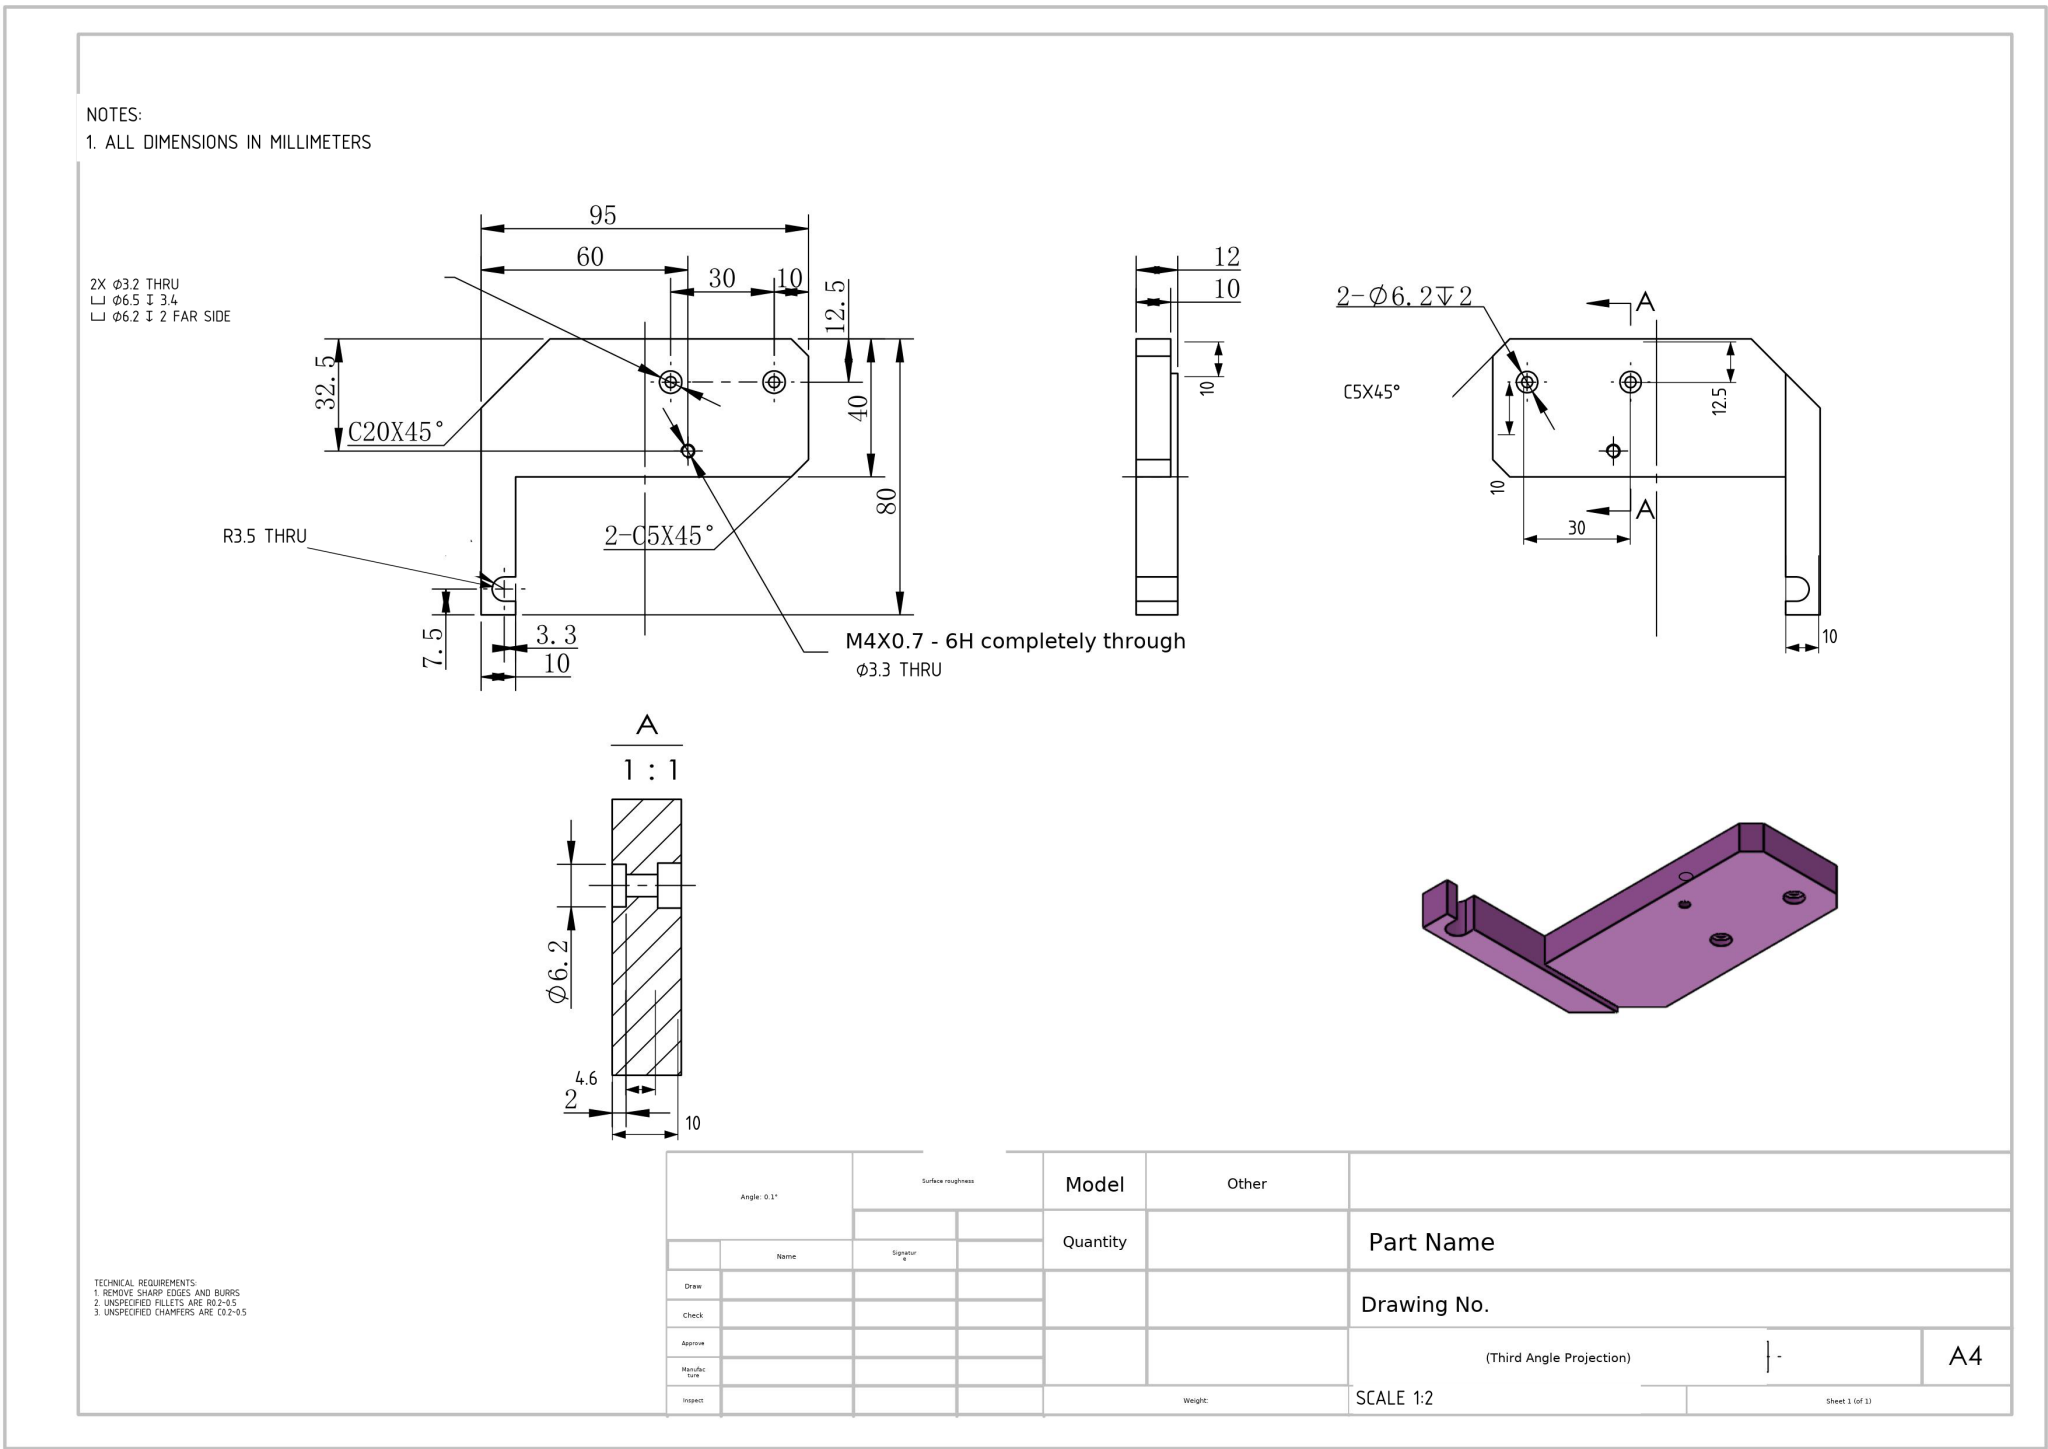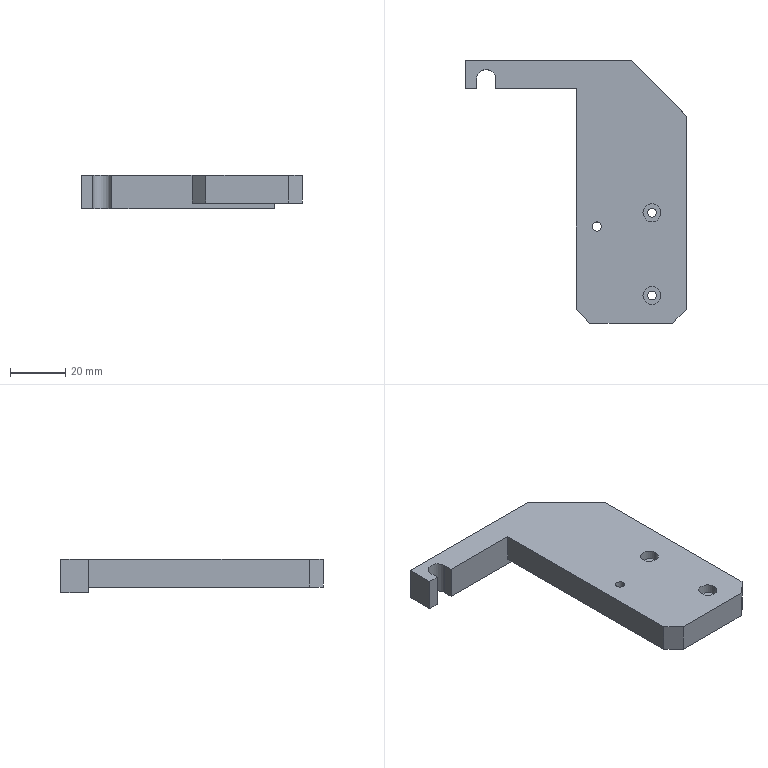Part | NX | mm | 1 solid | 34 faces | box 80 x 95 x 12 mm | volume 40036 mm3 | plane 19 | cylinder 15 | commonest cylinder face diameters 6.5 x4 3.2 x4 6.2 x4 3.3 x2 7 x1